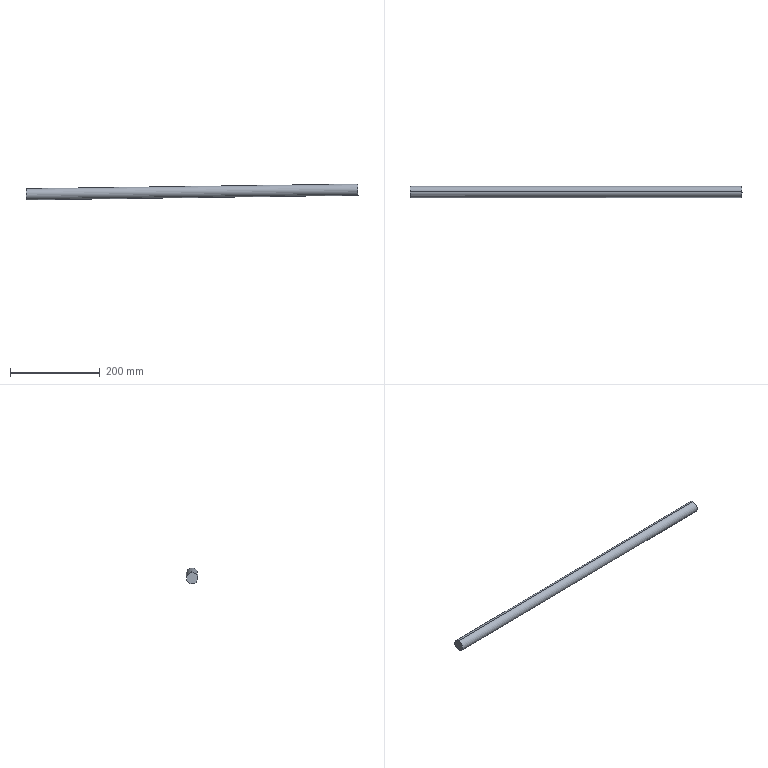Component | SolidWorks | DA-0220-Part15-1 | 1 solid | 4 faces | box 740.28 x 25.3 x 35.32 mm | volume 363247 mm3 | cylinder 2 | plane 2 | commonest cylinder face diameters 25 x2
build123d program:
from build123d import *

# Parameters (mm, degrees)
SKETCH1_R           = 12.5
BOSS_EXTRUDE1_DEPTH = 740


with BuildPart() as part:
    # Sketch1 → Boss-Extrude1 (new body)
    with BuildSketch(Plane.XY):
        Circle(SKETCH1_R)
    extrude(amount=BOSS_EXTRUDE1_DEPTH)


solid = part.part

# Placed as in the assembly
solid = solid.moved(Location((1035.898, -165.633, 463), (178.341, -89.2, -176.364)))
STEP:
#1=COLOUR_RGB('',0.7922,0.8196,0.9333);
#2=FILL_AREA_STYLE_COLOUR('',#1);
#3=FILL_AREA_STYLE('',(#2));
#4=SURFACE_STYLE_FILL_AREA(#3);
#5=SURFACE_SIDE_STYLE('',(#4));
#6=SURFACE_STYLE_USAGE(.BOTH.,#5);
#7=PRESENTATION_STYLE_ASSIGNMENT((#6));
#8=CARTESIAN_POINT('',(11.659,-6.562,17.331));
#9=VERTEX_POINT('',#8);
#10=CARTESIAN_POINT('',(11.645,-6.503,18.313));
#11=VERTEX_POINT('',#10);
#12=CARTESIAN_POINT('',(11.652,-6.533,17.822));
#13=DIRECTION('',(-0.9999,-0.000404,-0.01395));
#14=DIRECTION('',(0.01395,-0.05978,-0.9981));
#15=AXIS2_PLACEMENT_3D('',#12,#13,#14);
#16=CIRCLE('',#15,0.4921);
#17=EDGE_CURVE('',#9,#11,#16,.T.);
#18=ORIENTED_EDGE('',*,*,#17,.F.);
#19=CARTESIAN_POINT('',(40.79,-6.55,17.737));
#20=VERTEX_POINT('',#19);
#21=CARTESIAN_POINT('',(11.659,-6.562,17.331));
#22=DIRECTION('',(0.9999,0.000404,0.01395));
#23=VECTOR('',#22,39.37);
#24=LINE('',#21,#23);
#25=EDGE_CURVE('',#9,#20,#24,.T.);
#26=ORIENTED_EDGE('',*,*,#25,.T.);
#27=CARTESIAN_POINT('',(40.777,-6.492,18.72));
#28=VERTEX_POINT('',#27);
#29=CARTESIAN_POINT('',(40.783,-6.521,18.228));
#30=DIRECTION('',(-0.9999,-0.000404,-0.01395));
#31=DIRECTION('',(0.01395,-0.05978,-0.9981));
#32=AXIS2_PLACEMENT_3D('',#29,#30,#31);
#33=CIRCLE('',#32,0.4921);
#34=EDGE_CURVE('',#20,#28,#33,.T.);
#35=ORIENTED_EDGE('',*,*,#34,.T.);
#36=CARTESIAN_POINT('',(11.645,-6.503,18.313));
#37=DIRECTION('',(0.9999,0.000404,0.01395));
#38=VECTOR('',#37,39.37);
#39=LINE('',#36,#38);
#40=EDGE_CURVE('',#11,#28,#39,.T.);
#41=ORIENTED_EDGE('',*,*,#40,.F.);
#42=EDGE_LOOP('',(#18,#26,#35,#41));
#43=FACE_OUTER_BOUND('',#42,.T.);
#44=CARTESIAN_POINT('',(11.652,-6.533,17.822));
#45=DIRECTION('',(0.9999,0.000404,0.01395));
#46=DIRECTION('',(-0.01395,0.05978,0.9981));
#47=AXIS2_PLACEMENT_3D('',#44,#45,#46);
#48=CYLINDRICAL_SURFACE('',#47,0.4921);
#49=ADVANCED_FACE('',(#43),#48,.T.);
#50=ORIENTED_EDGE('',*,*,#25,.F.);
#51=CARTESIAN_POINT('',(11.652,-6.533,17.822));
#52=DIRECTION('',(-0.9999,-0.000404,-0.01395));
#53=DIRECTION('',(0.01395,-0.05978,-0.9981));
#54=AXIS2_PLACEMENT_3D('',#51,#52,#53);
#55=CIRCLE('',#54,0.4921);
#56=EDGE_CURVE('',#11,#9,#55,.T.);
#57=ORIENTED_EDGE('',*,*,#56,.F.);
#58=ORIENTED_EDGE('',*,*,#40,.T.);
#59=CARTESIAN_POINT('',(40.783,-6.521,18.228));
#60=DIRECTION('',(-0.9999,-0.000404,-0.01395));
#61=DIRECTION('',(0.01395,-0.05978,-0.9981));
#62=AXIS2_PLACEMENT_3D('',#59,#60,#61);
#63=CIRCLE('',#62,0.4921);
#64=EDGE_CURVE('',#28,#20,#63,.T.);
#65=ORIENTED_EDGE('',*,*,#64,.T.);
#66=EDGE_LOOP('',(#50,#57,#58,#65));
#67=FACE_OUTER_BOUND('',#66,.T.);
#68=CARTESIAN_POINT('',(11.652,-6.533,17.822));
#69=DIRECTION('',(0.9999,0.000404,0.01395));
#70=DIRECTION('',(-0.01395,0.05978,0.9981));
#71=AXIS2_PLACEMENT_3D('',#68,#69,#70);
#72=CYLINDRICAL_SURFACE('',#71,0.4921);
#73=ADVANCED_FACE('',(#67),#72,.T.);
#74=ORIENTED_EDGE('',*,*,#56,.T.);
#75=ORIENTED_EDGE('',*,*,#17,.T.);
#76=EDGE_LOOP('',(#74,#75));
#77=FACE_OUTER_BOUND('',#76,.T.);
#78=CARTESIAN_POINT('',(11.652,-6.533,17.822));
#79=DIRECTION('',(-0.9999,-0.000404,-0.01395));
#80=DIRECTION('',(0.01395,-0.05978,-0.9981));
#81=AXIS2_PLACEMENT_3D('',#78,#79,#80);
#82=PLANE('',#81);
#83=ADVANCED_FACE('',(#77),#82,.T.);
#84=ORIENTED_EDGE('',*,*,#64,.F.);
#85=ORIENTED_EDGE('',*,*,#34,.F.);
#86=EDGE_LOOP('',(#84,#85));
#87=FACE_OUTER_BOUND('',#86,.T.);
#88=CARTESIAN_POINT('',(40.783,-6.521,18.228));
#89=DIRECTION('',(-0.9999,-0.000404,-0.01395));
#90=DIRECTION('',(0.01395,-0.05978,-0.9981));
#91=AXIS2_PLACEMENT_3D('',#88,#89,#90);
#92=PLANE('',#91);
#93=ADVANCED_FACE('',(#87),#92,.F.);
#94=CLOSED_SHELL('',(#49,#73,#83,#93));
#95=MANIFOLD_SOLID_BREP('',#94);
#96=STYLED_ITEM('',(#7),#95);
#97=(LENGTH_UNIT()NAMED_UNIT(*)SI_UNIT($,.METRE.));
#98=LENGTH_MEASURE_WITH_UNIT(LENGTH_MEASURE(0.0254),#97);
#99=DIMENSIONAL_EXPONENTS(1.,0.,0.,0.,0.,0.,0.);
#100=(CONVERSION_BASED_UNIT('',#98)LENGTH_UNIT()NAMED_UNIT(#99));
#101=UNCERTAINTY_MEASURE_WITH_UNIT(LENGTH_MEASURE(0.00001),#100,'','');
#102=(NAMED_UNIT(*)PLANE_ANGLE_UNIT()SI_UNIT($,.RADIAN.));
#103=(NAMED_UNIT(*)SI_UNIT($,.STERADIAN.)SOLID_ANGLE_UNIT());
#104=(GEOMETRIC_REPRESENTATION_CONTEXT(3)GLOBAL_UNCERTAINTY_ASSIGNED_CONTEXT((#101))GLOBAL_UNIT_ASSIGNED_CONTEXT((#100,#102,#103))REPRESENTATION_CONTEXT('',''));
#105=MECHANICAL_DESIGN_GEOMETRIC_PRESENTATION_REPRESENTATION('',(#96),#104);
#106=CARTESIAN_POINT('',(0.,0.,0.));
#107=DIRECTION('',(0.,0.,1.));
#108=DIRECTION('',(1.,0.,0.));
#109=AXIS2_PLACEMENT_3D('',#106,#107,#108);
#110=(LENGTH_UNIT()NAMED_UNIT(*)SI_UNIT($,.METRE.));
#111=LENGTH_MEASURE_WITH_UNIT(LENGTH_MEASURE(0.0254),#110);
#112=DIMENSIONAL_EXPONENTS(1.,0.,0.,0.,0.,0.,0.);
#113=(CONVERSION_BASED_UNIT('',#111)LENGTH_UNIT()NAMED_UNIT(#112));
#114=UNCERTAINTY_MEASURE_WITH_UNIT(LENGTH_MEASURE(0.00001),#113,'','');
#115=(NAMED_UNIT(*)PLANE_ANGLE_UNIT()SI_UNIT($,.RADIAN.));
#116=(NAMED_UNIT(*)SI_UNIT($,.STERADIAN.)SOLID_ANGLE_UNIT());
#117=(GEOMETRIC_REPRESENTATION_CONTEXT(3)GLOBAL_UNCERTAINTY_ASSIGNED_CONTEXT((#114))GLOBAL_UNIT_ASSIGNED_CONTEXT((#113,#115,#116))REPRESENTATION_CONTEXT('',''));
#118=ADVANCED_BREP_SHAPE_REPRESENTATION('',(#95,#109),#117);
#119=PRESENTATION_LAYER_ASSIGNMENT('','',(#96));